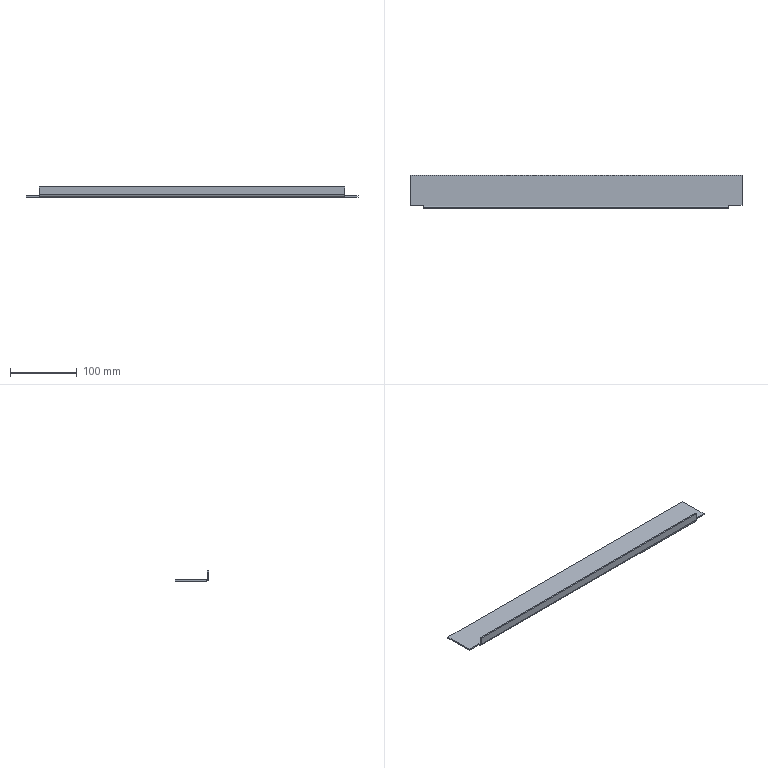Component | SolidWorks | RearRightSidePlateAssembly-1_RearRightSidePlateDoorHorizontalRib-2 | 1 solid | 18 faces | box 496 x 50 x 15 mm | volume 59882 mm3 | plane 16 | cylinder 2 | commonest cylinder face diameters 8 x1 4 x1 | material Plain Carbon Steel
STEP:
#1=COLOUR_RGB('',0.7922,0.8196,0.9333);
#2=FILL_AREA_STYLE_COLOUR('',#1);
#3=FILL_AREA_STYLE('',(#2));
#4=SURFACE_STYLE_FILL_AREA(#3);
#5=SURFACE_SIDE_STYLE('',(#4));
#6=SURFACE_STYLE_USAGE(.BOTH.,#5);
#7=PRESENTATION_STYLE_ASSIGNMENT((#6));
#8=CARTESIAN_POINT('',(96.35,47.699,36.515));
#9=VERTEX_POINT('',#8);
#10=CARTESIAN_POINT('',(96.35,47.778,36.515));
#11=VERTEX_POINT('',#10);
#12=CARTESIAN_POINT('',(96.35,47.699,36.515));
#13=DIRECTION('',(-0.,1.,0.));
#14=VECTOR('',#13,39.37);
#15=LINE('',#12,#14);
#16=EDGE_CURVE('',#9,#11,#15,.T.);
#17=ORIENTED_EDGE('',*,*,#16,.F.);
#18=CARTESIAN_POINT('',(96.35,47.856,36.357));
#19=VERTEX_POINT('',#18);
#20=CARTESIAN_POINT('',(96.35,47.856,36.515));
#21=DIRECTION('',(-1.,-0.,0.));
#22=DIRECTION('',(0.,0.,1.));
#23=AXIS2_PLACEMENT_3D('',#20,#21,#22);
#24=CIRCLE('',#23,0.1575);
#25=EDGE_CURVE('',#19,#9,#24,.T.);
#26=ORIENTED_EDGE('',*,*,#25,.F.);
#27=CARTESIAN_POINT('',(96.35,47.856,36.436));
#28=VERTEX_POINT('',#27);
#29=CARTESIAN_POINT('',(96.35,47.856,36.436));
#30=DIRECTION('',(-0.,0.,-1.));
#31=VECTOR('',#30,39.37);
#32=LINE('',#29,#31);
#33=EDGE_CURVE('',#28,#19,#32,.T.);
#34=ORIENTED_EDGE('',*,*,#33,.F.);
#35=CARTESIAN_POINT('',(96.35,47.856,36.515));
#36=DIRECTION('',(-1.,-0.,0.));
#37=DIRECTION('',(0.,0.,1.));
#38=AXIS2_PLACEMENT_3D('',#35,#36,#37);
#39=CIRCLE('',#38,0.07874);
#40=EDGE_CURVE('',#28,#11,#39,.T.);
#41=ORIENTED_EDGE('',*,*,#40,.T.);
#42=EDGE_LOOP('',(#17,#26,#34,#41));
#43=FACE_OUTER_BOUND('',#42,.T.);
#44=CARTESIAN_POINT('',(96.35,47.699,36.515));
#45=DIRECTION('',(1.,0.,-0.));
#46=DIRECTION('',(0.,-0.,1.));
#47=AXIS2_PLACEMENT_3D('',#44,#45,#46);
#48=PLANE('',#47);
#49=ADVANCED_FACE('',(#43),#48,.T.);
#50=CARTESIAN_POINT('',(96.35,47.699,36.948));
#51=VERTEX_POINT('',#50);
#52=CARTESIAN_POINT('',(96.35,47.699,36.357));
#53=DIRECTION('',(0.,-0.,1.));
#54=VECTOR('',#53,39.37);
#55=LINE('',#52,#54);
#56=EDGE_CURVE('',#9,#51,#55,.T.);
#57=ORIENTED_EDGE('',*,*,#56,.F.);
#58=ORIENTED_EDGE('',*,*,#16,.T.);
#59=CARTESIAN_POINT('',(96.35,47.778,36.948));
#60=VERTEX_POINT('',#59);
#61=CARTESIAN_POINT('',(96.35,47.778,36.357));
#62=DIRECTION('',(0.,-0.,1.));
#63=VECTOR('',#62,39.37);
#64=LINE('',#61,#63);
#65=EDGE_CURVE('',#11,#60,#64,.T.);
#66=ORIENTED_EDGE('',*,*,#65,.T.);
#67=CARTESIAN_POINT('',(96.35,47.699,36.948));
#68=DIRECTION('',(-0.,1.,0.));
#69=VECTOR('',#68,39.37);
#70=LINE('',#67,#69);
#71=EDGE_CURVE('',#51,#60,#70,.T.);
#72=ORIENTED_EDGE('',*,*,#71,.F.);
#73=EDGE_LOOP('',(#57,#58,#66,#72));
#74=FACE_OUTER_BOUND('',#73,.T.);
#75=CARTESIAN_POINT('',(96.35,47.856,36.436));
#76=DIRECTION('',(1.,0.,-0.));
#77=DIRECTION('',(0.,-0.,1.));
#78=AXIS2_PLACEMENT_3D('',#75,#76,#77);
#79=PLANE('',#78);
#80=ADVANCED_FACE('',(#74),#79,.T.);
#81=CARTESIAN_POINT('',(78.397,47.856,36.357));
#82=VERTEX_POINT('',#81);
#83=CARTESIAN_POINT('',(78.397,47.856,36.436));
#84=VERTEX_POINT('',#83);
#85=CARTESIAN_POINT('',(78.397,47.856,36.357));
#86=DIRECTION('',(0.,-0.,1.));
#87=VECTOR('',#86,39.37);
#88=LINE('',#85,#87);
#89=EDGE_CURVE('',#82,#84,#88,.T.);
#90=ORIENTED_EDGE('',*,*,#89,.F.);
#91=CARTESIAN_POINT('',(78.397,47.699,36.515));
#92=VERTEX_POINT('',#91);
#93=CARTESIAN_POINT('',(78.397,47.856,36.515));
#94=DIRECTION('',(-1.,-0.,0.));
#95=DIRECTION('',(0.,0.,1.));
#96=AXIS2_PLACEMENT_3D('',#93,#94,#95);
#97=CIRCLE('',#96,0.1575);
#98=EDGE_CURVE('',#82,#92,#97,.T.);
#99=ORIENTED_EDGE('',*,*,#98,.T.);
#100=CARTESIAN_POINT('',(78.397,47.778,36.515));
#101=VERTEX_POINT('',#100);
#102=CARTESIAN_POINT('',(78.397,47.778,36.515));
#103=DIRECTION('',(0.,-1.,-0.));
#104=VECTOR('',#103,39.37);
#105=LINE('',#102,#104);
#106=EDGE_CURVE('',#101,#92,#105,.T.);
#107=ORIENTED_EDGE('',*,*,#106,.F.);
#108=CARTESIAN_POINT('',(78.397,47.856,36.515));
#109=DIRECTION('',(-1.,-0.,0.));
#110=DIRECTION('',(0.,0.,1.));
#111=AXIS2_PLACEMENT_3D('',#108,#109,#110);
#112=CIRCLE('',#111,0.07874);
#113=EDGE_CURVE('',#84,#101,#112,.T.);
#114=ORIENTED_EDGE('',*,*,#113,.F.);
#115=EDGE_LOOP('',(#90,#99,#107,#114));
#116=FACE_OUTER_BOUND('',#115,.T.);
#117=CARTESIAN_POINT('',(78.397,47.856,36.357));
#118=DIRECTION('',(-1.,-0.,0.));
#119=DIRECTION('',(-0.,0.,-1.));
#120=AXIS2_PLACEMENT_3D('',#117,#118,#119);
#121=PLANE('',#120);
#122=ADVANCED_FACE('',(#116),#121,.T.);
#123=CARTESIAN_POINT('',(78.397,47.896,36.357));
#124=VERTEX_POINT('',#123);
#125=CARTESIAN_POINT('',(78.397,47.896,36.436));
#126=VERTEX_POINT('',#125);
#127=CARTESIAN_POINT('',(78.397,47.896,36.357));
#128=DIRECTION('',(0.,-0.,1.));
#129=VECTOR('',#128,39.37);
#130=LINE('',#127,#129);
#131=EDGE_CURVE('',#124,#126,#130,.T.);
#132=ORIENTED_EDGE('',*,*,#131,.F.);
#133=CARTESIAN_POINT('',(78.397,49.667,36.357));
#134=DIRECTION('',(0.,-1.,-0.));
#135=VECTOR('',#134,39.37);
#136=LINE('',#133,#135);
#137=EDGE_CURVE('',#124,#82,#136,.T.);
#138=ORIENTED_EDGE('',*,*,#137,.T.);
#139=ORIENTED_EDGE('',*,*,#89,.T.);
#140=CARTESIAN_POINT('',(78.397,49.667,36.436));
#141=DIRECTION('',(0.,-1.,-0.));
#142=VECTOR('',#141,39.37);
#143=LINE('',#140,#142);
#144=EDGE_CURVE('',#126,#84,#143,.T.);
#145=ORIENTED_EDGE('',*,*,#144,.F.);
#146=EDGE_LOOP('',(#132,#138,#139,#145));
#147=FACE_OUTER_BOUND('',#146,.T.);
#148=CARTESIAN_POINT('',(78.397,47.778,36.515));
#149=DIRECTION('',(-1.,-0.,0.));
#150=DIRECTION('',(-0.,0.,-1.));
#151=AXIS2_PLACEMENT_3D('',#148,#149,#150);
#152=PLANE('',#151);
#153=ADVANCED_FACE('',(#147),#152,.T.);
#154=CARTESIAN_POINT('',(78.397,47.778,36.948));
#155=VERTEX_POINT('',#154);
#156=CARTESIAN_POINT('',(78.397,47.778,36.357));
#157=DIRECTION('',(0.,-0.,1.));
#158=VECTOR('',#157,39.37);
#159=LINE('',#156,#158);
#160=EDGE_CURVE('',#101,#155,#159,.T.);
#161=ORIENTED_EDGE('',*,*,#160,.T.);
#162=CARTESIAN_POINT('',(96.35,47.778,36.948));
#163=DIRECTION('',(-1.,-0.,0.));
#164=VECTOR('',#163,39.37);
#165=LINE('',#162,#164);
#166=EDGE_CURVE('',#60,#155,#165,.T.);
#167=ORIENTED_EDGE('',*,*,#166,.F.);
#168=ORIENTED_EDGE('',*,*,#65,.F.);
#169=CARTESIAN_POINT('',(96.35,47.778,36.515));
#170=DIRECTION('',(-1.,-0.,0.));
#171=VECTOR('',#170,39.37);
#172=LINE('',#169,#171);
#173=EDGE_CURVE('',#11,#101,#172,.T.);
#174=ORIENTED_EDGE('',*,*,#173,.T.);
#175=EDGE_LOOP('',(#161,#167,#168,#174));
#176=FACE_OUTER_BOUND('',#175,.T.);
#177=CARTESIAN_POINT('',(96.35,47.778,36.357));
#178=DIRECTION('',(0.,-1.,-0.));
#179=DIRECTION('',(1.,0.,-0.));
#180=AXIS2_PLACEMENT_3D('',#177,#178,#179);
#181=PLANE('',#180);
#182=ADVANCED_FACE('',(#176),#181,.F.);
#183=CARTESIAN_POINT('',(78.397,47.699,36.948));
#184=VERTEX_POINT('',#183);
#185=CARTESIAN_POINT('',(78.397,47.699,36.948));
#186=DIRECTION('',(-0.,1.,0.));
#187=VECTOR('',#186,39.37);
#188=LINE('',#185,#187);
#189=EDGE_CURVE('',#184,#155,#188,.T.);
#190=ORIENTED_EDGE('',*,*,#189,.F.);
#191=CARTESIAN_POINT('',(96.35,47.699,36.948));
#192=DIRECTION('',(-1.,-0.,0.));
#193=VECTOR('',#192,39.37);
#194=LINE('',#191,#193);
#195=EDGE_CURVE('',#51,#184,#194,.T.);
#196=ORIENTED_EDGE('',*,*,#195,.F.);
#197=ORIENTED_EDGE('',*,*,#71,.T.);
#198=ORIENTED_EDGE('',*,*,#166,.T.);
#199=EDGE_LOOP('',(#190,#196,#197,#198));
#200=FACE_OUTER_BOUND('',#199,.T.);
#201=CARTESIAN_POINT('',(96.35,47.699,36.948));
#202=DIRECTION('',(0.,-0.,1.));
#203=DIRECTION('',(-1.,-0.,0.));
#204=AXIS2_PLACEMENT_3D('',#201,#202,#203);
#205=PLANE('',#204);
#206=ADVANCED_FACE('',(#200),#205,.T.);
#207=CARTESIAN_POINT('',(78.397,47.699,36.357));
#208=DIRECTION('',(0.,-0.,1.));
#209=VECTOR('',#208,39.37);
#210=LINE('',#207,#209);
#211=EDGE_CURVE('',#92,#184,#210,.T.);
#212=ORIENTED_EDGE('',*,*,#211,.F.);
#213=CARTESIAN_POINT('',(96.35,47.699,36.515));
#214=DIRECTION('',(-1.,-0.,0.));
#215=VECTOR('',#214,39.37);
#216=LINE('',#213,#215);
#217=EDGE_CURVE('',#9,#92,#216,.T.);
#218=ORIENTED_EDGE('',*,*,#217,.F.);
#219=ORIENTED_EDGE('',*,*,#56,.T.);
#220=ORIENTED_EDGE('',*,*,#195,.T.);
#221=EDGE_LOOP('',(#212,#218,#219,#220));
#222=FACE_OUTER_BOUND('',#221,.T.);
#223=CARTESIAN_POINT('',(96.35,47.699,36.357));
#224=DIRECTION('',(0.,-1.,-0.));
#225=DIRECTION('',(1.,0.,-0.));
#226=AXIS2_PLACEMENT_3D('',#223,#224,#225);
#227=PLANE('',#226);
#228=ADVANCED_FACE('',(#222),#227,.T.);
#229=ORIENTED_EDGE('',*,*,#98,.F.);
#230=CARTESIAN_POINT('',(96.35,47.856,36.357));
#231=DIRECTION('',(-1.,-0.,0.));
#232=VECTOR('',#231,39.37);
#233=LINE('',#230,#232);
#234=EDGE_CURVE('',#19,#82,#233,.T.);
#235=ORIENTED_EDGE('',*,*,#234,.F.);
#236=ORIENTED_EDGE('',*,*,#25,.T.);
#237=ORIENTED_EDGE('',*,*,#217,.T.);
#238=EDGE_LOOP('',(#229,#235,#236,#237));
#239=FACE_OUTER_BOUND('',#238,.T.);
#240=CARTESIAN_POINT('',(96.35,47.856,36.515));
#241=DIRECTION('',(-1.,-0.,0.));
#242=DIRECTION('',(0.,0.,-1.));
#243=AXIS2_PLACEMENT_3D('',#240,#241,#242);
#244=CYLINDRICAL_SURFACE('',#243,0.1575);
#245=ADVANCED_FACE('',(#239),#244,.T.);
#246=ORIENTED_EDGE('',*,*,#137,.F.);
#247=CARTESIAN_POINT('',(77.61,47.896,36.357));
#248=VERTEX_POINT('',#247);
#249=CARTESIAN_POINT('',(78.397,47.896,36.357));
#250=DIRECTION('',(1.,0.,-0.));
#251=VECTOR('',#250,39.37);
#252=LINE('',#249,#251);
#253=EDGE_CURVE('',#248,#124,#252,.T.);
#254=ORIENTED_EDGE('',*,*,#253,.F.);
#255=CARTESIAN_POINT('',(77.61,49.667,36.357));
#256=VERTEX_POINT('',#255);
#257=CARTESIAN_POINT('',(77.61,49.667,36.357));
#258=DIRECTION('',(0.,-1.,-0.));
#259=VECTOR('',#258,39.37);
#260=LINE('',#257,#259);
#261=EDGE_CURVE('',#256,#248,#260,.T.);
#262=ORIENTED_EDGE('',*,*,#261,.F.);
#263=CARTESIAN_POINT('',(97.137,49.667,36.357));
#264=VERTEX_POINT('',#263);
#265=CARTESIAN_POINT('',(96.35,49.667,36.357));
#266=DIRECTION('',(-1.,-0.,0.));
#267=VECTOR('',#266,39.37);
#268=LINE('',#265,#267);
#269=EDGE_CURVE('',#264,#256,#268,.T.);
#270=ORIENTED_EDGE('',*,*,#269,.F.);
#271=CARTESIAN_POINT('',(97.137,47.896,36.357));
#272=VERTEX_POINT('',#271);
#273=CARTESIAN_POINT('',(97.137,49.667,36.357));
#274=DIRECTION('',(-0.,1.,0.));
#275=VECTOR('',#274,39.37);
#276=LINE('',#273,#275);
#277=EDGE_CURVE('',#272,#264,#276,.T.);
#278=ORIENTED_EDGE('',*,*,#277,.F.);
#279=CARTESIAN_POINT('',(96.35,47.896,36.357));
#280=VERTEX_POINT('',#279);
#281=CARTESIAN_POINT('',(96.35,47.896,36.357));
#282=DIRECTION('',(1.,0.,-0.));
#283=VECTOR('',#282,39.37);
#284=LINE('',#281,#283);
#285=EDGE_CURVE('',#280,#272,#284,.T.);
#286=ORIENTED_EDGE('',*,*,#285,.F.);
#287=CARTESIAN_POINT('',(96.35,49.667,36.357));
#288=DIRECTION('',(0.,-1.,-0.));
#289=VECTOR('',#288,39.37);
#290=LINE('',#287,#289);
#291=EDGE_CURVE('',#280,#19,#290,.T.);
#292=ORIENTED_EDGE('',*,*,#291,.T.);
#293=ORIENTED_EDGE('',*,*,#234,.T.);
#294=EDGE_LOOP('',(#246,#254,#262,#270,#278,#286,#292,#293));
#295=FACE_OUTER_BOUND('',#294,.T.);
#296=CARTESIAN_POINT('',(96.35,49.667,36.357));
#297=DIRECTION('',(-0.,0.,-1.));
#298=DIRECTION('',(1.,0.,-0.));
#299=AXIS2_PLACEMENT_3D('',#296,#297,#298);
#300=PLANE('',#299);
#301=ADVANCED_FACE('',(#295),#300,.T.);
#302=ORIENTED_EDGE('',*,*,#269,.T.);
#303=CARTESIAN_POINT('',(77.61,49.667,36.436));
#304=VERTEX_POINT('',#303);
#305=CARTESIAN_POINT('',(77.61,49.667,36.357));
#306=DIRECTION('',(0.,-0.,1.));
#307=VECTOR('',#306,39.37);
#308=LINE('',#305,#307);
#309=EDGE_CURVE('',#256,#304,#308,.T.);
#310=ORIENTED_EDGE('',*,*,#309,.T.);
#311=CARTESIAN_POINT('',(97.137,49.667,36.436));
#312=VERTEX_POINT('',#311);
#313=CARTESIAN_POINT('',(96.35,49.667,36.436));
#314=DIRECTION('',(-1.,-0.,0.));
#315=VECTOR('',#314,39.37);
#316=LINE('',#313,#315);
#317=EDGE_CURVE('',#312,#304,#316,.T.);
#318=ORIENTED_EDGE('',*,*,#317,.F.);
#319=CARTESIAN_POINT('',(97.137,49.667,36.357));
#320=DIRECTION('',(0.,-0.,1.));
#321=VECTOR('',#320,39.37);
#322=LINE('',#319,#321);
#323=EDGE_CURVE('',#264,#312,#322,.T.);
#324=ORIENTED_EDGE('',*,*,#323,.F.);
#325=EDGE_LOOP('',(#302,#310,#318,#324));
#326=FACE_OUTER_BOUND('',#325,.T.);
#327=CARTESIAN_POINT('',(96.35,49.667,36.436));
#328=DIRECTION('',(-0.,1.,0.));
#329=DIRECTION('',(-1.,-0.,0.));
#330=AXIS2_PLACEMENT_3D('',#327,#328,#329);
#331=PLANE('',#330);
#332=ADVANCED_FACE('',(#326),#331,.T.);
#333=ORIENTED_EDGE('',*,*,#317,.T.);
#334=CARTESIAN_POINT('',(77.61,47.896,36.436));
#335=VERTEX_POINT('',#334);
#336=CARTESIAN_POINT('',(77.61,49.667,36.436));
#337=DIRECTION('',(0.,-1.,-0.));
#338=VECTOR('',#337,39.37);
#339=LINE('',#336,#338);
#340=EDGE_CURVE('',#304,#335,#339,.T.);
#341=ORIENTED_EDGE('',*,*,#340,.T.);
#342=CARTESIAN_POINT('',(78.397,47.896,36.436));
#343=DIRECTION('',(1.,0.,-0.));
#344=VECTOR('',#343,39.37);
#345=LINE('',#342,#344);
#346=EDGE_CURVE('',#335,#126,#345,.T.);
#347=ORIENTED_EDGE('',*,*,#346,.T.);
#348=ORIENTED_EDGE('',*,*,#144,.T.);
#349=CARTESIAN_POINT('',(96.35,47.856,36.436));
#350=DIRECTION('',(-1.,-0.,0.));
#351=VECTOR('',#350,39.37);
#352=LINE('',#349,#351);
#353=EDGE_CURVE('',#28,#84,#352,.T.);
#354=ORIENTED_EDGE('',*,*,#353,.F.);
#355=CARTESIAN_POINT('',(96.35,47.896,36.436));
#356=VERTEX_POINT('',#355);
#357=CARTESIAN_POINT('',(96.35,49.667,36.436));
#358=DIRECTION('',(0.,-1.,-0.));
#359=VECTOR('',#358,39.37);
#360=LINE('',#357,#359);
#361=EDGE_CURVE('',#356,#28,#360,.T.);
#362=ORIENTED_EDGE('',*,*,#361,.F.);
#363=CARTESIAN_POINT('',(97.137,47.896,36.436));
#364=VERTEX_POINT('',#363);
#365=CARTESIAN_POINT('',(96.35,47.896,36.436));
#366=DIRECTION('',(1.,0.,-0.));
#367=VECTOR('',#366,39.37);
#368=LINE('',#365,#367);
#369=EDGE_CURVE('',#356,#364,#368,.T.);
#370=ORIENTED_EDGE('',*,*,#369,.T.);
#371=CARTESIAN_POINT('',(97.137,49.667,36.436));
#372=DIRECTION('',(-0.,1.,0.));
#373=VECTOR('',#372,39.37);
#374=LINE('',#371,#373);
#375=EDGE_CURVE('',#364,#312,#374,.T.);
#376=ORIENTED_EDGE('',*,*,#375,.T.);
#377=EDGE_LOOP('',(#333,#341,#347,#348,#354,#362,#370,#376));
#378=FACE_OUTER_BOUND('',#377,.T.);
#379=CARTESIAN_POINT('',(96.35,49.667,36.436));
#380=DIRECTION('',(-0.,0.,-1.));
#381=DIRECTION('',(1.,0.,-0.));
#382=AXIS2_PLACEMENT_3D('',#379,#380,#381);
#383=PLANE('',#382);
#384=ADVANCED_FACE('',(#378),#383,.F.);
#385=ORIENTED_EDGE('',*,*,#113,.T.);
#386=ORIENTED_EDGE('',*,*,#173,.F.);
#387=ORIENTED_EDGE('',*,*,#40,.F.);
#388=ORIENTED_EDGE('',*,*,#353,.T.);
#389=EDGE_LOOP('',(#385,#386,#387,#388));
#390=FACE_OUTER_BOUND('',#389,.T.);
#391=CARTESIAN_POINT('',(96.35,47.856,36.515));
#392=DIRECTION('',(-1.,-0.,0.));
#393=DIRECTION('',(0.,0.,-1.));
#394=AXIS2_PLACEMENT_3D('',#391,#392,#393);
#395=CYLINDRICAL_SURFACE('',#394,0.07874);
#396=ADVANCED_FACE('',(#390),#395,.F.);
#397=CARTESIAN_POINT('',(96.35,47.896,36.357));
#398=DIRECTION('',(0.,-0.,1.));
#399=VECTOR('',#398,39.37);
#400=LINE('',#397,#399);
#401=EDGE_CURVE('',#280,#356,#400,.T.);
#402=ORIENTED_EDGE('',*,*,#401,.T.);
#403=ORIENTED_EDGE('',*,*,#361,.T.);
#404=ORIENTED_EDGE('',*,*,#33,.T.);
#405=ORIENTED_EDGE('',*,*,#291,.F.);
#406=EDGE_LOOP('',(#402,#403,#404,#405));
#407=FACE_OUTER_BOUND('',#406,.T.);
#408=CARTESIAN_POINT('',(96.35,47.856,36.515));
#409=DIRECTION('',(1.,0.,-0.));
#410=DIRECTION('',(0.,-0.,1.));
#411=AXIS2_PLACEMENT_3D('',#408,#409,#410);
#412=PLANE('',#411);
#413=ADVANCED_FACE('',(#407),#412,.T.);
#414=ORIENTED_EDGE('',*,*,#160,.F.);
#415=ORIENTED_EDGE('',*,*,#106,.T.);
#416=ORIENTED_EDGE('',*,*,#211,.T.);
#417=ORIENTED_EDGE('',*,*,#189,.T.);
#418=EDGE_LOOP('',(#414,#415,#416,#417));
#419=FACE_OUTER_BOUND('',#418,.T.);
#420=CARTESIAN_POINT('',(78.397,47.856,36.515));
#421=DIRECTION('',(1.,0.,-0.));
#422=DIRECTION('',(0.,-0.,1.));
#423=AXIS2_PLACEMENT_3D('',#420,#421,#422);
#424=PLANE('',#423);
#425=ADVANCED_FACE('',(#419),#424,.F.);
#426=ORIENTED_EDGE('',*,*,#375,.F.);
#427=CARTESIAN_POINT('',(97.137,47.896,36.357));
#428=DIRECTION('',(0.,-0.,1.));
#429=VECTOR('',#428,39.37);
#430=LINE('',#427,#429);
#431=EDGE_CURVE('',#272,#364,#430,.T.);
#432=ORIENTED_EDGE('',*,*,#431,.F.);
#433=ORIENTED_EDGE('',*,*,#277,.T.);
#434=ORIENTED_EDGE('',*,*,#323,.T.);
#435=EDGE_LOOP('',(#426,#432,#433,#434));
#436=FACE_OUTER_BOUND('',#435,.T.);
#437=CARTESIAN_POINT('',(97.137,49.667,36.357));
#438=DIRECTION('',(1.,0.,-0.));
#439=DIRECTION('',(0.,-0.,1.));
#440=AXIS2_PLACEMENT_3D('',#437,#438,#439);
#441=PLANE('',#440);
#442=ADVANCED_FACE('',(#436),#441,.T.);
#443=ORIENTED_EDGE('',*,*,#369,.F.);
#444=ORIENTED_EDGE('',*,*,#401,.F.);
#445=ORIENTED_EDGE('',*,*,#285,.T.);
#446=ORIENTED_EDGE('',*,*,#431,.T.);
#447=EDGE_LOOP('',(#443,#444,#445,#446));
#448=FACE_OUTER_BOUND('',#447,.T.);
#449=CARTESIAN_POINT('',(96.35,47.896,36.357));
#450=DIRECTION('',(0.,-1.,-0.));
#451=DIRECTION('',(1.,0.,-0.));
#452=AXIS2_PLACEMENT_3D('',#449,#450,#451);
#453=PLANE('',#452);
#454=ADVANCED_FACE('',(#448),#453,.T.);
#455=ORIENTED_EDGE('',*,*,#346,.F.);
#456=CARTESIAN_POINT('',(77.61,47.896,36.357));
#457=DIRECTION('',(0.,-0.,1.));
#458=VECTOR('',#457,39.37);
#459=LINE('',#456,#458);
#460=EDGE_CURVE('',#248,#335,#459,.T.);
#461=ORIENTED_EDGE('',*,*,#460,.F.);
#462=ORIENTED_EDGE('',*,*,#253,.T.);
#463=ORIENTED_EDGE('',*,*,#131,.T.);
#464=EDGE_LOOP('',(#455,#461,#462,#463));
#465=FACE_OUTER_BOUND('',#464,.T.);
#466=CARTESIAN_POINT('',(78.397,47.896,36.357));
#467=DIRECTION('',(0.,-1.,-0.));
#468=DIRECTION('',(1.,0.,-0.));
#469=AXIS2_PLACEMENT_3D('',#466,#467,#468);
#470=PLANE('',#469);
#471=ADVANCED_FACE('',(#465),#470,.T.);
#472=ORIENTED_EDGE('',*,*,#340,.F.);
#473=ORIENTED_EDGE('',*,*,#309,.F.);
#474=ORIENTED_EDGE('',*,*,#261,.T.);
#475=ORIENTED_EDGE('',*,*,#460,.T.);
#476=EDGE_LOOP('',(#472,#473,#474,#475));
#477=FACE_OUTER_BOUND('',#476,.T.);
#478=CARTESIAN_POINT('',(77.61,49.667,36.357));
#479=DIRECTION('',(-1.,-0.,0.));
#480=DIRECTION('',(-0.,0.,-1.));
#481=AXIS2_PLACEMENT_3D('',#478,#479,#480);
#482=PLANE('',#481);
#483=ADVANCED_FACE('',(#477),#482,.T.);
#484=CLOSED_SHELL('',(#49,#80,#122,#153,#182,#206,#228,#245,#301,#332,#384,#396,#413,#425,#442,#454,#471,#483));
#485=MANIFOLD_SOLID_BREP('',#484);
#486=STYLED_ITEM('',(#7),#485);
#487=PRESENTATION_LAYER_ASSIGNMENT('','',(#486));
#488=CARTESIAN_POINT('',(0.,0.,0.));
#489=DIRECTION('',(0.,0.,1.));
#490=DIRECTION('',(1.,0.,0.));
#491=AXIS2_PLACEMENT_3D('',#488,#489,#490);
#492=(LENGTH_UNIT()NAMED_UNIT(*)SI_UNIT($,.METRE.));
#493=LENGTH_MEASURE_WITH_UNIT(LENGTH_MEASURE(0.0254),#492);
#494=DIMENSIONAL_EXPONENTS(1.,0.,0.,0.,0.,0.,0.);
#495=(CONVERSION_BASED_UNIT('',#493)LENGTH_UNIT()NAMED_UNIT(#494));
#496=UNCERTAINTY_MEASURE_WITH_UNIT(LENGTH_MEASURE(0.00001),#495,'','');
#497=(NAMED_UNIT(*)PLANE_ANGLE_UNIT()SI_UNIT($,.RADIAN.));
#498=(NAMED_UNIT(*)SI_UNIT($,.STERADIAN.)SOLID_ANGLE_UNIT());
#499=(GEOMETRIC_REPRESENTATION_CONTEXT(3)GLOBAL_UNCERTAINTY_ASSIGNED_CONTEXT((#496))GLOBAL_UNIT_ASSIGNED_CONTEXT((#495,#497,#498))REPRESENTATION_CONTEXT('',''));
#500=ADVANCED_BREP_SHAPE_REPRESENTATION('',(#485,#491),#499);
#501=(LENGTH_UNIT()NAMED_UNIT(*)SI_UNIT($,.METRE.));
#502=LENGTH_MEASURE_WITH_UNIT(LENGTH_MEASURE(0.0254),#501);
#503=DIMENSIONAL_EXPONENTS(1.,0.,0.,0.,0.,0.,0.);
#504=(CONVERSION_BASED_UNIT('',#502)LENGTH_UNIT()NAMED_UNIT(#503));
#505=UNCERTAINTY_MEASURE_WITH_UNIT(LENGTH_MEASURE(0.00001),#504,'','');
#506=(NAMED_UNIT(*)PLANE_ANGLE_UNIT()SI_UNIT($,.RADIAN.));
#507=(NAMED_UNIT(*)SI_UNIT($,.STERADIAN.)SOLID_ANGLE_UNIT());
#508=(GEOMETRIC_REPRESENTATION_CONTEXT(3)GLOBAL_UNCERTAINTY_ASSIGNED_CONTEXT((#505))GLOBAL_UNIT_ASSIGNED_CONTEXT((#504,#506,#507))REPRESENTATION_CONTEXT('',''));
#509=MECHANICAL_DESIGN_GEOMETRIC_PRESENTATION_REPRESENTATION('',(#486),#508);